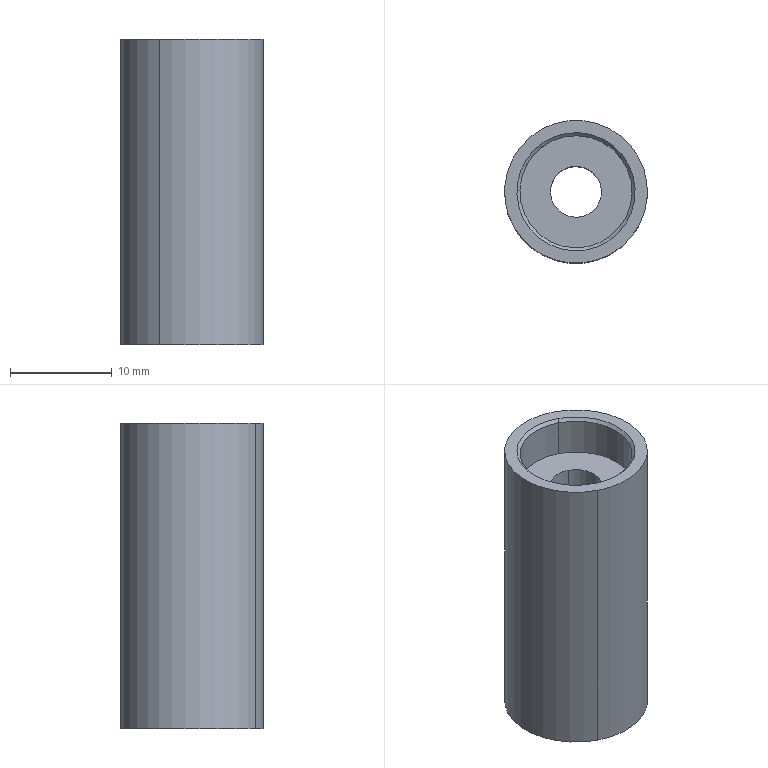Component | SolidWorks | AdhesiveRoller-1 | 1 solid | 16 faces | box 14 x 14 x 30 mm | volume 3423 mm3 | cylinder 8 | cone 4 | plane 4 | commonest cylinder face diameters 11 x4 14 x2 5 x2
STEP:
#1=COLOUR_RGB('',0.7922,0.8196,0.9333);
#2=FILL_AREA_STYLE_COLOUR('',#1);
#3=FILL_AREA_STYLE('',(#2));
#4=SURFACE_STYLE_FILL_AREA(#3);
#5=SURFACE_SIDE_STYLE('',(#4));
#6=SURFACE_STYLE_USAGE(.BOTH.,#5);
#7=PRESENTATION_STYLE_ASSIGNMENT((#6));
#8=CARTESIAN_POINT('',(-6.49,3.211,1.935));
#9=VERTEX_POINT('',#8);
#10=CARTESIAN_POINT('',(-6.238,3.7,1.935));
#11=VERTEX_POINT('',#10);
#12=CARTESIAN_POINT('',(-6.364,3.455,1.935));
#13=DIRECTION('',(-0.,0.,-1.));
#14=DIRECTION('',(-0.4581,-0.8889,0.));
#15=AXIS2_PLACEMENT_3D('',#12,#13,#14);
#16=CIRCLE('',#15,0.2756);
#17=EDGE_CURVE('',#9,#11,#16,.T.);
#18=ORIENTED_EDGE('',*,*,#17,.T.);
#19=CARTESIAN_POINT('',(-6.238,3.7,0.7536));
#20=VERTEX_POINT('',#19);
#21=CARTESIAN_POINT('',(-6.238,3.7,1.935));
#22=DIRECTION('',(-0.,0.,-1.));
#23=VECTOR('',#22,39.37);
#24=LINE('',#21,#23);
#25=EDGE_CURVE('',#11,#20,#24,.T.);
#26=ORIENTED_EDGE('',*,*,#25,.T.);
#27=CARTESIAN_POINT('',(-6.49,3.211,0.7536));
#28=VERTEX_POINT('',#27);
#29=CARTESIAN_POINT('',(-6.364,3.455,0.7536));
#30=DIRECTION('',(0.,-0.,1.));
#31=DIRECTION('',(-0.4581,-0.8889,0.));
#32=AXIS2_PLACEMENT_3D('',#29,#30,#31);
#33=CIRCLE('',#32,0.2756);
#34=EDGE_CURVE('',#20,#28,#33,.T.);
#35=ORIENTED_EDGE('',*,*,#34,.T.);
#36=CARTESIAN_POINT('',(-6.49,3.211,1.935));
#37=DIRECTION('',(-0.,0.,-1.));
#38=VECTOR('',#37,39.37);
#39=LINE('',#36,#38);
#40=EDGE_CURVE('',#9,#28,#39,.T.);
#41=ORIENTED_EDGE('',*,*,#40,.F.);
#42=EDGE_LOOP('',(#18,#26,#35,#41));
#43=FACE_OUTER_BOUND('',#42,.T.);
#44=CARTESIAN_POINT('',(-6.364,3.455,1.935));
#45=DIRECTION('',(-0.,0.,-1.));
#46=DIRECTION('',(-0.4581,-0.8889,0.));
#47=AXIS2_PLACEMENT_3D('',#44,#45,#46);
#48=CYLINDRICAL_SURFACE('',#47,0.2756);
#49=ADVANCED_FACE('',(#43),#48,.T.);
#50=CARTESIAN_POINT('',(-6.265,3.648,0.7654));
#51=VERTEX_POINT('',#50);
#52=CARTESIAN_POINT('',(-6.463,3.263,0.7654));
#53=VERTEX_POINT('',#52);
#54=CARTESIAN_POINT('',(-6.364,3.455,0.7654));
#55=DIRECTION('',(-0.,0.,-1.));
#56=DIRECTION('',(-0.4581,-0.8889,0.));
#57=AXIS2_PLACEMENT_3D('',#54,#55,#56);
#58=CIRCLE('',#57,0.2165);
#59=EDGE_CURVE('',#51,#53,#58,.T.);
#60=ORIENTED_EDGE('',*,*,#59,.F.);
#61=CARTESIAN_POINT('',(-6.259,3.658,0.7536));
#62=VERTEX_POINT('',#61);
#63=CARTESIAN_POINT('',(-6.259,3.658,0.7536));
#64=DIRECTION('',(0.3239,0.6285,-0.7071));
#65=VECTOR('',#64,39.37);
#66=LINE('',#63,#65);
#67=EDGE_CURVE('',#51,#62,#66,.T.);
#68=ORIENTED_EDGE('',*,*,#67,.T.);
#69=CARTESIAN_POINT('',(-6.469,3.253,0.7536));
#70=VERTEX_POINT('',#69);
#71=CARTESIAN_POINT('',(-6.364,3.455,0.7536));
#72=DIRECTION('',(-0.,0.,-1.));
#73=DIRECTION('',(-0.4581,-0.8889,0.));
#74=AXIS2_PLACEMENT_3D('',#71,#72,#73);
#75=CIRCLE('',#74,0.2283);
#76=EDGE_CURVE('',#62,#70,#75,.T.);
#77=ORIENTED_EDGE('',*,*,#76,.T.);
#78=CARTESIAN_POINT('',(-6.469,3.253,0.7536));
#79=DIRECTION('',(-0.3239,-0.6285,-0.7071));
#80=VECTOR('',#79,39.37);
#81=LINE('',#78,#80);
#82=EDGE_CURVE('',#53,#70,#81,.T.);
#83=ORIENTED_EDGE('',*,*,#82,.F.);
#84=EDGE_LOOP('',(#60,#68,#77,#83));
#85=FACE_OUTER_BOUND('',#84,.T.);
#86=CARTESIAN_POINT('',(-6.364,3.455,0.7536));
#87=DIRECTION('',(-0.,0.,-1.));
#88=DIRECTION('',(-0.4581,-0.8889,0.));
#89=AXIS2_PLACEMENT_3D('',#86,#87,#88);
#90=CONICAL_SURFACE('',#89,0.2283,0.7854);
#91=ADVANCED_FACE('',(#85),#90,.F.);
#92=CARTESIAN_POINT('',(-6.463,3.263,1.923));
#93=VERTEX_POINT('',#92);
#94=CARTESIAN_POINT('',(-6.265,3.648,1.923));
#95=VERTEX_POINT('',#94);
#96=CARTESIAN_POINT('',(-6.364,3.455,1.923));
#97=DIRECTION('',(0.,-0.,1.));
#98=DIRECTION('',(0.4581,0.8889,0.));
#99=AXIS2_PLACEMENT_3D('',#96,#97,#98);
#100=CIRCLE('',#99,0.2165);
#101=EDGE_CURVE('',#93,#95,#100,.T.);
#102=ORIENTED_EDGE('',*,*,#101,.F.);
#103=CARTESIAN_POINT('',(-6.469,3.253,1.935));
#104=VERTEX_POINT('',#103);
#105=CARTESIAN_POINT('',(-6.469,3.253,1.935));
#106=DIRECTION('',(-0.3239,-0.6285,0.7071));
#107=VECTOR('',#106,39.37);
#108=LINE('',#105,#107);
#109=EDGE_CURVE('',#93,#104,#108,.T.);
#110=ORIENTED_EDGE('',*,*,#109,.T.);
#111=CARTESIAN_POINT('',(-6.259,3.658,1.935));
#112=VERTEX_POINT('',#111);
#113=CARTESIAN_POINT('',(-6.364,3.455,1.935));
#114=DIRECTION('',(-0.,0.,-1.));
#115=DIRECTION('',(0.4581,0.8889,0.));
#116=AXIS2_PLACEMENT_3D('',#113,#114,#115);
#117=CIRCLE('',#116,0.2283);
#118=EDGE_CURVE('',#112,#104,#117,.T.);
#119=ORIENTED_EDGE('',*,*,#118,.F.);
#120=CARTESIAN_POINT('',(-6.259,3.658,1.935));
#121=DIRECTION('',(0.3239,0.6285,0.7071));
#122=VECTOR('',#121,39.37);
#123=LINE('',#120,#122);
#124=EDGE_CURVE('',#95,#112,#123,.T.);
#125=ORIENTED_EDGE('',*,*,#124,.F.);
#126=EDGE_LOOP('',(#102,#110,#119,#125));
#127=FACE_OUTER_BOUND('',#126,.T.);
#128=CARTESIAN_POINT('',(-6.364,3.455,1.935));
#129=DIRECTION('',(0.,-0.,1.));
#130=DIRECTION('',(0.4581,0.8889,0.));
#131=AXIS2_PLACEMENT_3D('',#128,#129,#130);
#132=CONICAL_SURFACE('',#131,0.2283,0.7854);
#133=ADVANCED_FACE('',(#127),#132,.F.);
#134=CARTESIAN_POINT('',(-6.265,3.648,0.911));
#135=VERTEX_POINT('',#134);
#136=CARTESIAN_POINT('',(-6.463,3.263,0.911));
#137=VERTEX_POINT('',#136);
#138=CARTESIAN_POINT('',(-6.364,3.455,0.911));
#139=DIRECTION('',(-0.,0.,-1.));
#140=DIRECTION('',(-0.4581,-0.8889,0.));
#141=AXIS2_PLACEMENT_3D('',#138,#139,#140);
#142=CIRCLE('',#141,0.2165);
#143=EDGE_CURVE('',#135,#137,#142,.T.);
#144=ORIENTED_EDGE('',*,*,#143,.F.);
#145=CARTESIAN_POINT('',(-6.265,3.648,0.911));
#146=DIRECTION('',(-0.,0.,-1.));
#147=VECTOR('',#146,39.37);
#148=LINE('',#145,#147);
#149=EDGE_CURVE('',#135,#51,#148,.T.);
#150=ORIENTED_EDGE('',*,*,#149,.T.);
#151=ORIENTED_EDGE('',*,*,#59,.T.);
#152=CARTESIAN_POINT('',(-6.463,3.263,0.911));
#153=DIRECTION('',(-0.,0.,-1.));
#154=VECTOR('',#153,39.37);
#155=LINE('',#152,#154);
#156=EDGE_CURVE('',#137,#53,#155,.T.);
#157=ORIENTED_EDGE('',*,*,#156,.F.);
#158=EDGE_LOOP('',(#144,#150,#151,#157));
#159=FACE_OUTER_BOUND('',#158,.T.);
#160=CARTESIAN_POINT('',(-6.364,3.455,0.911));
#161=DIRECTION('',(-0.,0.,-1.));
#162=DIRECTION('',(-0.4581,-0.8889,0.));
#163=AXIS2_PLACEMENT_3D('',#160,#161,#162);
#164=CYLINDRICAL_SURFACE('',#163,0.2165);
#165=ADVANCED_FACE('',(#159),#164,.F.);
#166=CARTESIAN_POINT('',(-6.463,3.263,1.777));
#167=VERTEX_POINT('',#166);
#168=CARTESIAN_POINT('',(-6.265,3.648,1.777));
#169=VERTEX_POINT('',#168);
#170=CARTESIAN_POINT('',(-6.364,3.455,1.777));
#171=DIRECTION('',(0.,-0.,1.));
#172=DIRECTION('',(0.4581,0.8889,0.));
#173=AXIS2_PLACEMENT_3D('',#170,#171,#172);
#174=CIRCLE('',#173,0.2165);
#175=EDGE_CURVE('',#167,#169,#174,.T.);
#176=ORIENTED_EDGE('',*,*,#175,.F.);
#177=CARTESIAN_POINT('',(-6.463,3.263,1.777));
#178=DIRECTION('',(0.,-0.,1.));
#179=VECTOR('',#178,39.37);
#180=LINE('',#177,#179);
#181=EDGE_CURVE('',#167,#93,#180,.T.);
#182=ORIENTED_EDGE('',*,*,#181,.T.);
#183=ORIENTED_EDGE('',*,*,#101,.T.);
#184=CARTESIAN_POINT('',(-6.265,3.648,1.777));
#185=DIRECTION('',(0.,-0.,1.));
#186=VECTOR('',#185,39.37);
#187=LINE('',#184,#186);
#188=EDGE_CURVE('',#169,#95,#187,.T.);
#189=ORIENTED_EDGE('',*,*,#188,.F.);
#190=EDGE_LOOP('',(#176,#182,#183,#189));
#191=FACE_OUTER_BOUND('',#190,.T.);
#192=CARTESIAN_POINT('',(-6.364,3.455,1.777));
#193=DIRECTION('',(0.,-0.,1.));
#194=DIRECTION('',(0.4581,0.8889,0.));
#195=AXIS2_PLACEMENT_3D('',#192,#193,#194);
#196=CYLINDRICAL_SURFACE('',#195,0.2165);
#197=ADVANCED_FACE('',(#191),#196,.F.);
#198=CARTESIAN_POINT('',(-6.319,3.543,1.777));
#199=VERTEX_POINT('',#198);
#200=CARTESIAN_POINT('',(-6.409,3.368,1.777));
#201=VERTEX_POINT('',#200);
#202=CARTESIAN_POINT('',(-6.364,3.455,1.777));
#203=DIRECTION('',(-0.,0.,-1.));
#204=DIRECTION('',(-0.4581,-0.8889,0.));
#205=AXIS2_PLACEMENT_3D('',#202,#203,#204);
#206=CIRCLE('',#205,0.09843);
#207=EDGE_CURVE('',#199,#201,#206,.T.);
#208=ORIENTED_EDGE('',*,*,#207,.F.);
#209=CARTESIAN_POINT('',(-6.319,3.543,0.911));
#210=VERTEX_POINT('',#209);
#211=CARTESIAN_POINT('',(-6.319,3.543,1.935));
#212=DIRECTION('',(-0.,0.,-1.));
#213=VECTOR('',#212,39.37);
#214=LINE('',#211,#213);
#215=EDGE_CURVE('',#199,#210,#214,.T.);
#216=ORIENTED_EDGE('',*,*,#215,.T.);
#217=CARTESIAN_POINT('',(-6.409,3.368,0.911));
#218=VERTEX_POINT('',#217);
#219=CARTESIAN_POINT('',(-6.364,3.455,0.911));
#220=DIRECTION('',(0.,-0.,1.));
#221=DIRECTION('',(-0.4581,-0.8889,0.));
#222=AXIS2_PLACEMENT_3D('',#219,#220,#221);
#223=CIRCLE('',#222,0.09843);
#224=EDGE_CURVE('',#218,#210,#223,.T.);
#225=ORIENTED_EDGE('',*,*,#224,.F.);
#226=CARTESIAN_POINT('',(-6.409,3.368,1.935));
#227=DIRECTION('',(-0.,0.,-1.));
#228=VECTOR('',#227,39.37);
#229=LINE('',#226,#228);
#230=EDGE_CURVE('',#201,#218,#229,.T.);
#231=ORIENTED_EDGE('',*,*,#230,.F.);
#232=EDGE_LOOP('',(#208,#216,#225,#231));
#233=FACE_OUTER_BOUND('',#232,.T.);
#234=CARTESIAN_POINT('',(-6.364,3.455,1.935));
#235=DIRECTION('',(-0.,0.,-1.));
#236=DIRECTION('',(-0.4581,-0.8889,0.));
#237=AXIS2_PLACEMENT_3D('',#234,#235,#236);
#238=CYLINDRICAL_SURFACE('',#237,0.09843);
#239=ADVANCED_FACE('',(#233),#238,.F.);
#240=ORIENTED_EDGE('',*,*,#25,.F.);
#241=CARTESIAN_POINT('',(-6.364,3.455,1.935));
#242=DIRECTION('',(-0.,0.,-1.));
#243=DIRECTION('',(-0.4581,-0.8889,0.));
#244=AXIS2_PLACEMENT_3D('',#241,#242,#243);
#245=CIRCLE('',#244,0.2756);
#246=EDGE_CURVE('',#11,#9,#245,.T.);
#247=ORIENTED_EDGE('',*,*,#246,.T.);
#248=ORIENTED_EDGE('',*,*,#40,.T.);
#249=CARTESIAN_POINT('',(-6.364,3.455,0.7536));
#250=DIRECTION('',(0.,-0.,1.));
#251=DIRECTION('',(-0.4581,-0.8889,0.));
#252=AXIS2_PLACEMENT_3D('',#249,#250,#251);
#253=CIRCLE('',#252,0.2756);
#254=EDGE_CURVE('',#28,#20,#253,.T.);
#255=ORIENTED_EDGE('',*,*,#254,.T.);
#256=EDGE_LOOP('',(#240,#247,#248,#255));
#257=FACE_OUTER_BOUND('',#256,.T.);
#258=CARTESIAN_POINT('',(-6.364,3.455,1.935));
#259=DIRECTION('',(-0.,0.,-1.));
#260=DIRECTION('',(-0.4581,-0.8889,0.));
#261=AXIS2_PLACEMENT_3D('',#258,#259,#260);
#262=CYLINDRICAL_SURFACE('',#261,0.2756);
#263=ADVANCED_FACE('',(#257),#262,.T.);
#264=ORIENTED_EDGE('',*,*,#254,.F.);
#265=ORIENTED_EDGE('',*,*,#34,.F.);
#266=EDGE_LOOP('',(#264,#265));
#267=FACE_OUTER_BOUND('',#266,.T.);
#268=CARTESIAN_POINT('',(-6.364,3.455,0.7536));
#269=DIRECTION('',(-0.,0.,-1.));
#270=DIRECTION('',(-0.4581,-0.8889,0.));
#271=AXIS2_PLACEMENT_3D('',#268,#269,#270);
#272=CIRCLE('',#271,0.2283);
#273=EDGE_CURVE('',#70,#62,#272,.T.);
#274=ORIENTED_EDGE('',*,*,#273,.F.);
#275=ORIENTED_EDGE('',*,*,#76,.F.);
#276=EDGE_LOOP('',(#274,#275));
#277=FACE_BOUND('',#276,.T.);
#278=CARTESIAN_POINT('',(-6.364,3.455,0.7536));
#279=DIRECTION('',(0.,-0.,1.));
#280=DIRECTION('',(0.4581,0.8889,0.));
#281=AXIS2_PLACEMENT_3D('',#278,#279,#280);
#282=PLANE('',#281);
#283=ADVANCED_FACE('',(#267,#277),#282,.F.);
#284=ORIENTED_EDGE('',*,*,#17,.F.);
#285=ORIENTED_EDGE('',*,*,#246,.F.);
#286=EDGE_LOOP('',(#284,#285));
#287=FACE_OUTER_BOUND('',#286,.T.);
#288=ORIENTED_EDGE('',*,*,#118,.T.);
#289=CARTESIAN_POINT('',(-6.364,3.455,1.935));
#290=DIRECTION('',(-0.,0.,-1.));
#291=DIRECTION('',(0.4581,0.8889,0.));
#292=AXIS2_PLACEMENT_3D('',#289,#290,#291);
#293=CIRCLE('',#292,0.2283);
#294=EDGE_CURVE('',#104,#112,#293,.T.);
#295=ORIENTED_EDGE('',*,*,#294,.T.);
#296=EDGE_LOOP('',(#288,#295));
#297=FACE_BOUND('',#296,.T.);
#298=CARTESIAN_POINT('',(-6.364,3.455,1.935));
#299=DIRECTION('',(0.,-0.,1.));
#300=DIRECTION('',(0.4581,0.8889,0.));
#301=AXIS2_PLACEMENT_3D('',#298,#299,#300);
#302=PLANE('',#301);
#303=ADVANCED_FACE('',(#287,#297),#302,.T.);
#304=ORIENTED_EDGE('',*,*,#67,.F.);
#305=CARTESIAN_POINT('',(-6.364,3.455,0.7654));
#306=DIRECTION('',(-0.,0.,-1.));
#307=DIRECTION('',(-0.4581,-0.8889,0.));
#308=AXIS2_PLACEMENT_3D('',#305,#306,#307);
#309=CIRCLE('',#308,0.2165);
#310=EDGE_CURVE('',#53,#51,#309,.T.);
#311=ORIENTED_EDGE('',*,*,#310,.F.);
#312=ORIENTED_EDGE('',*,*,#82,.T.);
#313=ORIENTED_EDGE('',*,*,#273,.T.);
#314=EDGE_LOOP('',(#304,#311,#312,#313));
#315=FACE_OUTER_BOUND('',#314,.T.);
#316=CARTESIAN_POINT('',(-6.364,3.455,0.7536));
#317=DIRECTION('',(-0.,0.,-1.));
#318=DIRECTION('',(-0.4581,-0.8889,0.));
#319=AXIS2_PLACEMENT_3D('',#316,#317,#318);
#320=CONICAL_SURFACE('',#319,0.2283,0.7854);
#321=ADVANCED_FACE('',(#315),#320,.F.);
#322=ORIENTED_EDGE('',*,*,#109,.F.);
#323=CARTESIAN_POINT('',(-6.364,3.455,1.923));
#324=DIRECTION('',(0.,-0.,1.));
#325=DIRECTION('',(0.4581,0.8889,0.));
#326=AXIS2_PLACEMENT_3D('',#323,#324,#325);
#327=CIRCLE('',#326,0.2165);
#328=EDGE_CURVE('',#95,#93,#327,.T.);
#329=ORIENTED_EDGE('',*,*,#328,.F.);
#330=ORIENTED_EDGE('',*,*,#124,.T.);
#331=ORIENTED_EDGE('',*,*,#294,.F.);
#332=EDGE_LOOP('',(#322,#329,#330,#331));
#333=FACE_OUTER_BOUND('',#332,.T.);
#334=CARTESIAN_POINT('',(-6.364,3.455,1.935));
#335=DIRECTION('',(0.,-0.,1.));
#336=DIRECTION('',(0.4581,0.8889,0.));
#337=AXIS2_PLACEMENT_3D('',#334,#335,#336);
#338=CONICAL_SURFACE('',#337,0.2283,0.7854);
#339=ADVANCED_FACE('',(#333),#338,.F.);
#340=ORIENTED_EDGE('',*,*,#149,.F.);
#341=CARTESIAN_POINT('',(-6.364,3.455,0.911));
#342=DIRECTION('',(-0.,0.,-1.));
#343=DIRECTION('',(-0.4581,-0.8889,0.));
#344=AXIS2_PLACEMENT_3D('',#341,#342,#343);
#345=CIRCLE('',#344,0.2165);
#346=EDGE_CURVE('',#137,#135,#345,.T.);
#347=ORIENTED_EDGE('',*,*,#346,.F.);
#348=ORIENTED_EDGE('',*,*,#156,.T.);
#349=ORIENTED_EDGE('',*,*,#310,.T.);
#350=EDGE_LOOP('',(#340,#347,#348,#349));
#351=FACE_OUTER_BOUND('',#350,.T.);
#352=CARTESIAN_POINT('',(-6.364,3.455,0.911));
#353=DIRECTION('',(-0.,0.,-1.));
#354=DIRECTION('',(-0.4581,-0.8889,0.));
#355=AXIS2_PLACEMENT_3D('',#352,#353,#354);
#356=CYLINDRICAL_SURFACE('',#355,0.2165);
#357=ADVANCED_FACE('',(#351),#356,.F.);
#358=ORIENTED_EDGE('',*,*,#181,.F.);
#359=CARTESIAN_POINT('',(-6.364,3.455,1.777));
#360=DIRECTION('',(0.,-0.,1.));
#361=DIRECTION('',(0.4581,0.8889,0.));
#362=AXIS2_PLACEMENT_3D('',#359,#360,#361);
#363=CIRCLE('',#362,0.2165);
#364=EDGE_CURVE('',#169,#167,#363,.T.);
#365=ORIENTED_EDGE('',*,*,#364,.F.);
#366=ORIENTED_EDGE('',*,*,#188,.T.);
#367=ORIENTED_EDGE('',*,*,#328,.T.);
#368=EDGE_LOOP('',(#358,#365,#366,#367));
#369=FACE_OUTER_BOUND('',#368,.T.);
#370=CARTESIAN_POINT('',(-6.364,3.455,1.777));
#371=DIRECTION('',(0.,-0.,1.));
#372=DIRECTION('',(0.4581,0.8889,0.));
#373=AXIS2_PLACEMENT_3D('',#370,#371,#372);
#374=CYLINDRICAL_SURFACE('',#373,0.2165);
#375=ADVANCED_FACE('',(#369),#374,.F.);
#376=ORIENTED_EDGE('',*,*,#346,.T.);
#377=ORIENTED_EDGE('',*,*,#143,.T.);
#378=EDGE_LOOP('',(#376,#377));
#379=FACE_OUTER_BOUND('',#378,.T.);
#380=ORIENTED_EDGE('',*,*,#224,.T.);
#381=CARTESIAN_POINT('',(-6.364,3.455,0.911));
#382=DIRECTION('',(0.,-0.,1.));
#383=DIRECTION('',(-0.4581,-0.8889,0.));
#384=AXIS2_PLACEMENT_3D('',#381,#382,#383);
#385=CIRCLE('',#384,0.09843);
#386=EDGE_CURVE('',#210,#218,#385,.T.);
#387=ORIENTED_EDGE('',*,*,#386,.T.);
#388=EDGE_LOOP('',(#380,#387));
#389=FACE_BOUND('',#388,.T.);
#390=CARTESIAN_POINT('',(-6.364,3.455,0.911));
#391=DIRECTION('',(-0.,0.,-1.));
#392=DIRECTION('',(-0.4581,-0.8889,-0.));
#393=AXIS2_PLACEMENT_3D('',#390,#391,#392);
#394=PLANE('',#393);
#395=ADVANCED_FACE('',(#379,#389),#394,.T.);
#396=ORIENTED_EDGE('',*,*,#364,.T.);
#397=ORIENTED_EDGE('',*,*,#175,.T.);
#398=EDGE_LOOP('',(#396,#397));
#399=FACE_OUTER_BOUND('',#398,.T.);
#400=CARTESIAN_POINT('',(-6.364,3.455,1.777));
#401=DIRECTION('',(-0.,0.,-1.));
#402=DIRECTION('',(-0.4581,-0.8889,0.));
#403=AXIS2_PLACEMENT_3D('',#400,#401,#402);
#404=CIRCLE('',#403,0.09843);
#405=EDGE_CURVE('',#201,#199,#404,.T.);
#406=ORIENTED_EDGE('',*,*,#405,.T.);
#407=ORIENTED_EDGE('',*,*,#207,.T.);
#408=EDGE_LOOP('',(#406,#407));
#409=FACE_BOUND('',#408,.T.);
#410=CARTESIAN_POINT('',(-6.364,3.455,1.777));
#411=DIRECTION('',(0.,-0.,1.));
#412=DIRECTION('',(0.4581,0.8889,0.));
#413=AXIS2_PLACEMENT_3D('',#410,#411,#412);
#414=PLANE('',#413);
#415=ADVANCED_FACE('',(#399,#409),#414,.T.);
#416=ORIENTED_EDGE('',*,*,#215,.F.);
#417=ORIENTED_EDGE('',*,*,#405,.F.);
#418=ORIENTED_EDGE('',*,*,#230,.T.);
#419=ORIENTED_EDGE('',*,*,#386,.F.);
#420=EDGE_LOOP('',(#416,#417,#418,#419));
#421=FACE_OUTER_BOUND('',#420,.T.);
#422=CARTESIAN_POINT('',(-6.364,3.455,1.935));
#423=DIRECTION('',(-0.,0.,-1.));
#424=DIRECTION('',(-0.4581,-0.8889,0.));
#425=AXIS2_PLACEMENT_3D('',#422,#423,#424);
#426=CYLINDRICAL_SURFACE('',#425,0.09843);
#427=ADVANCED_FACE('',(#421),#426,.F.);
#428=CLOSED_SHELL('',(#49,#91,#133,#165,#197,#239,#263,#283,#303,#321,#339,#357,#375,#395,#415,#427));
#429=MANIFOLD_SOLID_BREP('',#428);
#430=STYLED_ITEM('',(#7),#429);
#431=(LENGTH_UNIT()NAMED_UNIT(*)SI_UNIT($,.METRE.));
#432=LENGTH_MEASURE_WITH_UNIT(LENGTH_MEASURE(0.0254),#431);
#433=DIMENSIONAL_EXPONENTS(1.,0.,0.,0.,0.,0.,0.);
#434=(CONVERSION_BASED_UNIT('',#432)LENGTH_UNIT()NAMED_UNIT(#433));
#435=UNCERTAINTY_MEASURE_WITH_UNIT(LENGTH_MEASURE(0.00001),#434,'','');
#436=(NAMED_UNIT(*)PLANE_ANGLE_UNIT()SI_UNIT($,.RADIAN.));
#437=(NAMED_UNIT(*)SI_UNIT($,.STERADIAN.)SOLID_ANGLE_UNIT());
#438=(GEOMETRIC_REPRESENTATION_CONTEXT(3)GLOBAL_UNCERTAINTY_ASSIGNED_CONTEXT((#435))GLOBAL_UNIT_ASSIGNED_CONTEXT((#434,#436,#437))REPRESENTATION_CONTEXT('',''));
#439=MECHANICAL_DESIGN_GEOMETRIC_PRESENTATION_REPRESENTATION('',(#430),#438);
#440=PRESENTATION_LAYER_ASSIGNMENT('','',(#430));
#441=CARTESIAN_POINT('',(0.,0.,0.));
#442=DIRECTION('',(0.,0.,1.));
#443=DIRECTION('',(1.,0.,0.));
#444=AXIS2_PLACEMENT_3D('',#441,#442,#443);
#445=(LENGTH_UNIT()NAMED_UNIT(*)SI_UNIT($,.METRE.));
#446=LENGTH_MEASURE_WITH_UNIT(LENGTH_MEASURE(0.0254),#445);
#447=DIMENSIONAL_EXPONENTS(1.,0.,0.,0.,0.,0.,0.);
#448=(CONVERSION_BASED_UNIT('',#446)LENGTH_UNIT()NAMED_UNIT(#447));
#449=UNCERTAINTY_MEASURE_WITH_UNIT(LENGTH_MEASURE(0.00001),#448,'','');
#450=(NAMED_UNIT(*)PLANE_ANGLE_UNIT()SI_UNIT($,.RADIAN.));
#451=(NAMED_UNIT(*)SI_UNIT($,.STERADIAN.)SOLID_ANGLE_UNIT());
#452=(GEOMETRIC_REPRESENTATION_CONTEXT(3)GLOBAL_UNCERTAINTY_ASSIGNED_CONTEXT((#449))GLOBAL_UNIT_ASSIGNED_CONTEXT((#448,#450,#451))REPRESENTATION_CONTEXT('',''));
#453=ADVANCED_BREP_SHAPE_REPRESENTATION('',(#429,#444),#452);